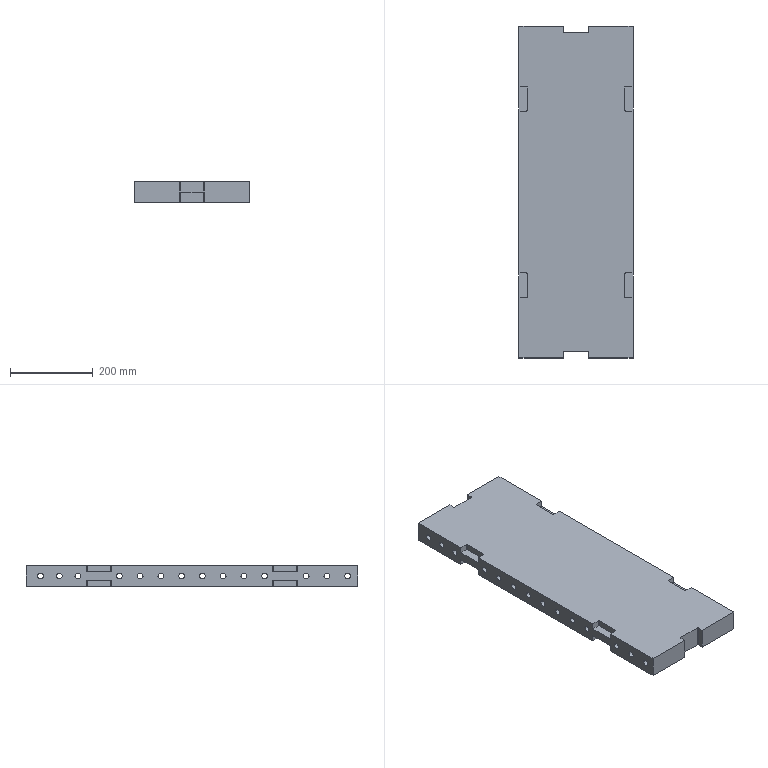Component | SolidWorks | Part5-1 | 1 solid | 94 faces | volume 10173716 mm3 | cylinder 48 | plane 46 | commonest cylinder face diameters 14 x28 4 x20